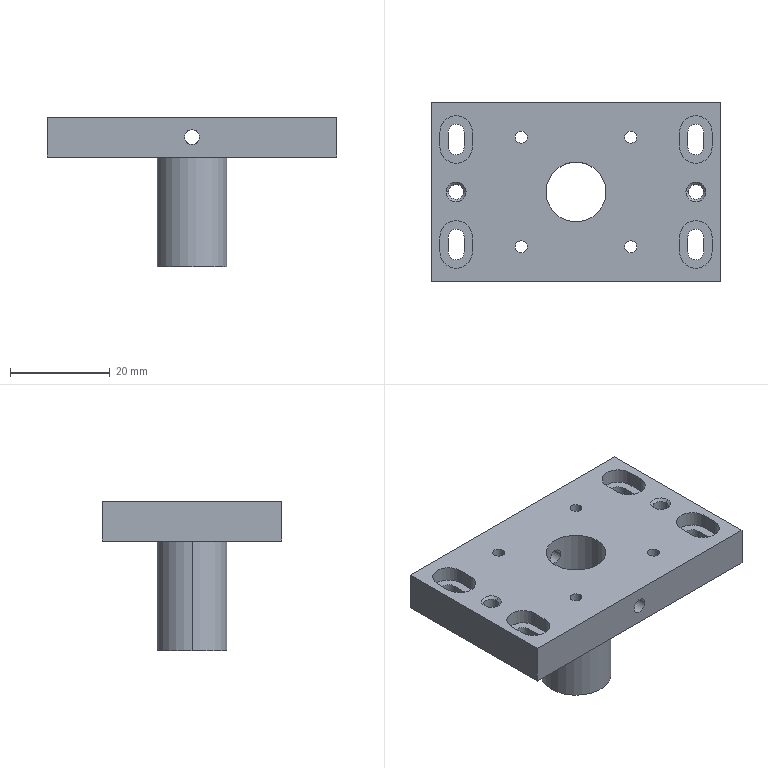Component | SolidWorks | MotorAssemblyWhen2-1_37bi-mpp70-3020-1 | 1 solid | 71 faces | volume 15279 mm3 | cylinder 36 | plane 27 | cone 8 | commonest cylinder face diameters 3 x8 2.4 x8 6.5 x8 3.2 x8 14 x2 12 x2